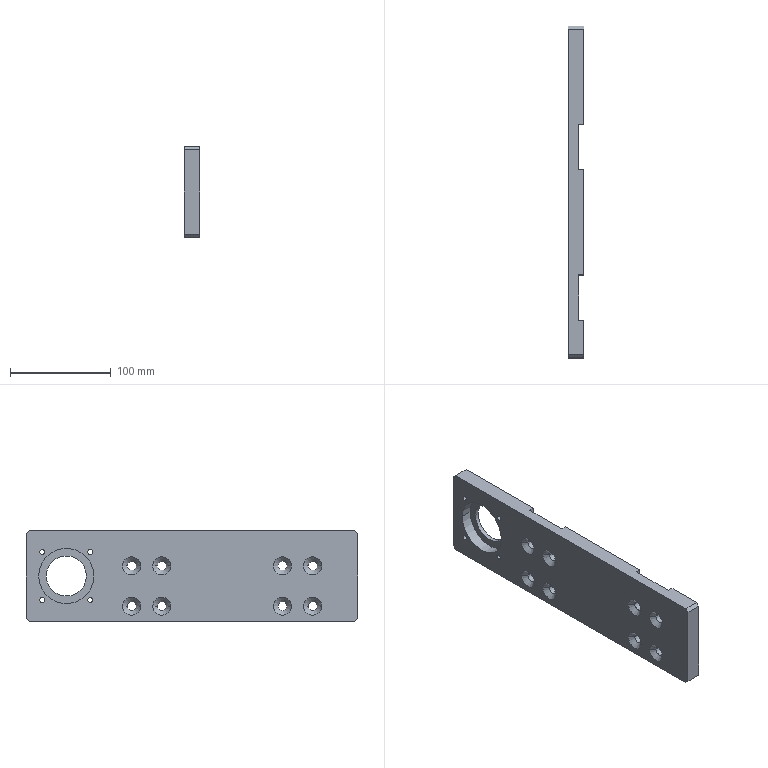Component | SolidWorks | LowerSideBeltXG-XG1-1_LowerSliderConnectingPlateXG-XG1-1 | 1 solid | 71 faces | box 15 x 330 x 90 mm | volume 363115 mm3 | cylinder 32 | cone 20 | plane 19 | commonest cylinder face diameters 9 x16 5 x8 6.8 x4 55 x2 40 x2
build123d program:
from build123d import *

# Parameters (mm, degrees)
SKETCH1_W                                            = 330
SKETCH1_H                                            = 90
BOSS_EXTRUDE1_DEPTH                                  = 7.5
TAPERED_COUNTERSUNK_HOLE_FOR_M8_HEXAGON_D            = 9
TAPERED_COUNTERSUNK_HOLE_FOR_M8_HEXAGON_CSINK_D      = 17.92
TAPERED_COUNTERSUNK_HOLE_FOR_M8_HEXAGON_CSINK_ANGLE  = 90
LPATTERN1_COUNT                                      = 2
LPATTERN1_PITCH                                      = 30
LPATTERN1_COUNT_DIR2                                 = 2
LPATTERN1_PITCH_DIR2                                 = 40
COUNTERSUNK_HOLE_2_FOR_M8_HEX_SOCKET_COU_D           = 9
COUNTERSUNK_HOLE_2_FOR_M8_HEX_SOCKET_COU_CSINK_D     = 17.92
COUNTERSUNK_HOLE_2_FOR_M8_HEX_SOCKET_COU_CSINK_ANGLE = 90
LPATTERN2_COUNT                                      = 2
LPATTERN2_PITCH                                      = 30
LPATTERN2_COUNT_DIR2                                 = 2
LPATTERN2_PITCH_DIR2                                 = 40
SKETCH6_R                                            = 20
CUT_EXTRUDE1_DEPTH                                   = 15
M6_TAPPED_HOLE1_D                                    = 5
CIRPATTERN1_COUNT                                    = 4
CHAMFER1_SIZE                                        = 3
M8_TAPPED_HOLE1_D                                    = 6.8
M8_TAPPED_HOLE1_DEPTH                                = 15.75
M8_TAPPED_HOLE1_TIP                                  = 2.043
SKETCH11_W                                           = 45
SKETCH11_H                                           = 16.654
SKETCH11_H_2                                         = 18.244
CUT_EXTRUDE2_DEPTH                                   = 189.099
SKETCH12_R                                           = 27.5
CUT_EXTRUDE3_DEPTH                                   = 11


with BuildPart() as part:
    # Sketch1 → Boss-Extrude1 (new, symmetric)
    with BuildSketch(Plane.XY):
        Rectangle(SKETCH1_W, SKETCH1_H)
    extrude(amount=BOSS_EXTRUDE1_DEPTH, both=True)

    # Tapered Countersunk Hole for M8 Hexagon (through all)
    with Locations(Plane(origin=(0, 0, -7.5), x_dir=(1, 0, 0), z_dir=(0, 0, -1))):
        with Locations((-90, -10)):
            tapered_countersunk_hole_for_m8_hexagon = CounterSinkHole(TAPERED_COUNTERSUNK_HOLE_FOR_M8_HEXAGON_D / 2, TAPERED_COUNTERSUNK_HOLE_FOR_M8_HEXAGON_CSINK_D / 2, counter_sink_angle=TAPERED_COUNTERSUNK_HOLE_FOR_M8_HEXAGON_CSINK_ANGLE)

    # LPattern1: Tapered Countersunk Hole for M8 Hexagon 2 × 2
    with Locations(*[(-i * LPATTERN1_PITCH, -j * LPATTERN1_PITCH_DIR2, 0) for i in range(LPATTERN1_COUNT) for j in range(LPATTERN1_COUNT_DIR2) if (i, j) != (0, 0)]):
        add(tapered_countersunk_hole_for_m8_hexagon, mode=Mode.SUBTRACT)

    # Countersunk Hole 2 for M8 Hex Socket Cou (through all)
    with Locations(Plane(origin=(0, 0, -7.5), x_dir=(1, 0, 0), z_dir=(0, 0, -1))):
        with Locations((60, -10)):
            countersunk_hole_2_for_m8_hex_socket_cou = CounterSinkHole(COUNTERSUNK_HOLE_2_FOR_M8_HEX_SOCKET_COU_D / 2, COUNTERSUNK_HOLE_2_FOR_M8_HEX_SOCKET_COU_CSINK_D / 2, counter_sink_angle=COUNTERSUNK_HOLE_2_FOR_M8_HEX_SOCKET_COU_CSINK_ANGLE)

    # LPattern2: Countersunk Hole 2 for M8 Hex Socket Cou 2 × 2
    with Locations(*[(-i * LPATTERN2_PITCH, -j * LPATTERN2_PITCH_DIR2, 0) for i in range(LPATTERN2_COUNT) for j in range(LPATTERN2_COUNT_DIR2) if (i, j) != (0, 0)]):
        add(countersunk_hole_2_for_m8_hex_socket_cou, mode=Mode.SUBTRACT)

    # Sketch6 → Cut-Extrude1 (cut)
    with BuildSketch(Plane.XY.offset(7.5)):
        with Locations((125, 0)):
            Circle(SKETCH6_R)
    extrude(amount=-CUT_EXTRUDE1_DEPTH, mode=Mode.SUBTRACT)

    # M6 Tapped Hole1 (through all)
    with Locations(Plane.XY.offset(7.5)):
        with Locations((101.135, 23.865)):
            m6_tapped_hole1 = Hole(M6_TAPPED_HOLE1_D / 2)

    # CirPattern1: M6 Tapped Hole1 ×4 about axis
    cirpattern1_axis = Axis((125, 0, 0), (0, 0, 1))
    for i in range(1, CIRPATTERN1_COUNT):
        add(m6_tapped_hole1.rotate(cirpattern1_axis, i * 360 / CIRPATTERN1_COUNT), mode=Mode.SUBTRACT)

    # Chamfer1
    chamfer1_edges = [part.edges().sort_by_distance(p)[0] for p in [
        (165, -45, 0),
        (-165, -45, 0),
        (-165, 45, 0),
        (165, 45, 0),
    ]]
    chamfer(chamfer1_edges, length=CHAMFER1_SIZE)

    # M8 Tapped Hole1
    with Locations(Plane.XZ.offset(45)):
        with Locations((-45, 0), (-15, 0)):
            Hole(M8_TAPPED_HOLE1_D / 2, depth=M8_TAPPED_HOLE1_DEPTH)
            with Locations((0, 0, -(M8_TAPPED_HOLE1_DEPTH + M8_TAPPED_HOLE1_TIP / 2))):  # 118° drill point
                Cone(0, M8_TAPPED_HOLE1_D / 2, M8_TAPPED_HOLE1_TIP, mode=Mode.SUBTRACT)

    # Sketch11 → Cut-Extrude2 (cut, through all)
    with BuildSketch(Plane(origin=(0, 45, 0), x_dir=(1, 0, 0), z_dir=(0, 1, 0))):
        with Locations((-105, -10.827)):
            Rectangle(SKETCH11_W, SKETCH11_H)
        with Locations((45, -11.622)):
            Rectangle(SKETCH11_W, SKETCH11_H_2)
    extrude(amount=-CUT_EXTRUDE2_DEPTH, mode=Mode.SUBTRACT)

    # Sketch12 → Cut-Extrude3 (cut)
    with BuildSketch(Plane(origin=(0, 0, -7.5), x_dir=(-1, 0, 0), z_dir=(0, 0, -1))):
        with Locations((-125, 0)):
            Circle(SKETCH12_R)
    extrude(amount=-CUT_EXTRUDE3_DEPTH, mode=Mode.SUBTRACT)


solid = part.part

# Placed as in the assembly
solid = solid.moved(Location((-373.72, 500, 114), (90, 90, 0)))